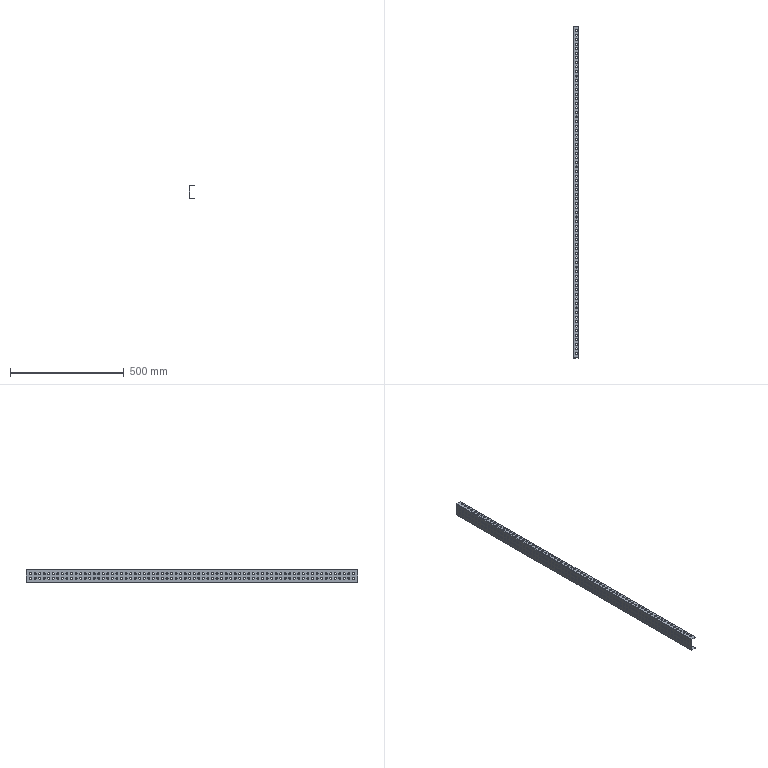Component | SolidWorks | KSHE-016.009-2 | 1 solid | 598 faces | volume 270119 mm3 | cylinder 580 | plane 18 | commonest cylinder face diameters 9 x576 4.2 x2 0.2 x2